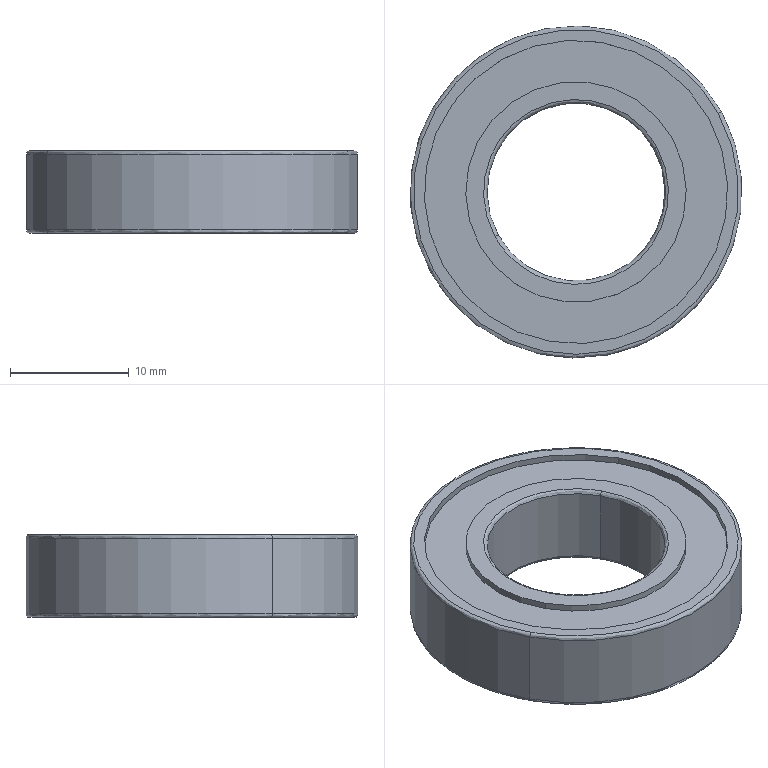Component | SolidWorks | LD101-02-B6902zz(D15xD28x7)-2-1 | 1 solid | 26 faces | volume 2801 mm3 | cylinder 12 | spline 8 | plane 6 | commonest cylinder face diameters 25.6 x4 18.6 x4 28 x2 15 x2 | material 60Si2Mn